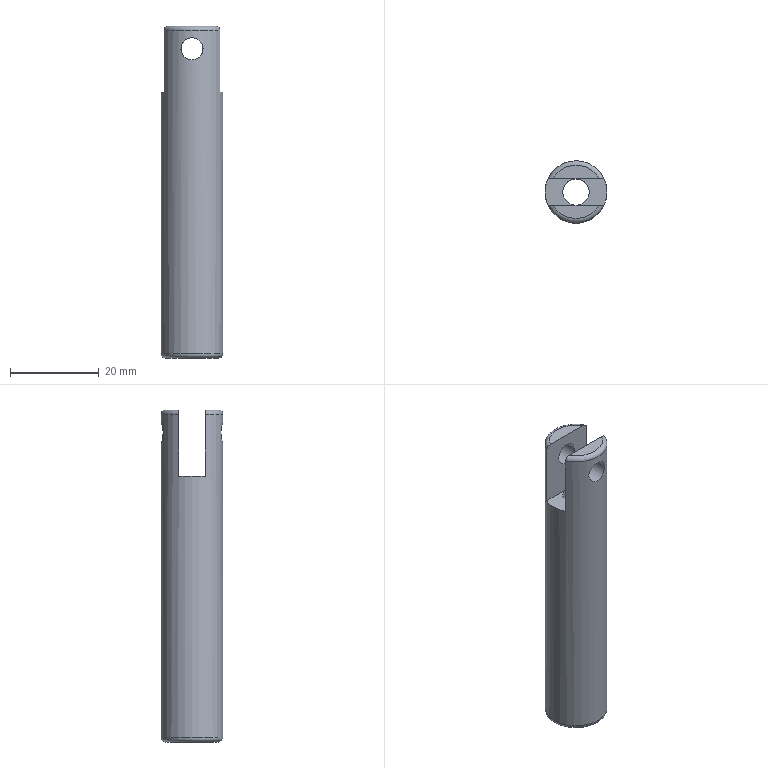Component | NX | CENTRE_ROD | 1 solid | 14 faces | volume 8460 mm3 | plane 7 | cylinder 4 | torus 3 | commonest cylinder face diameters 5 x2 14 x1 6 x1